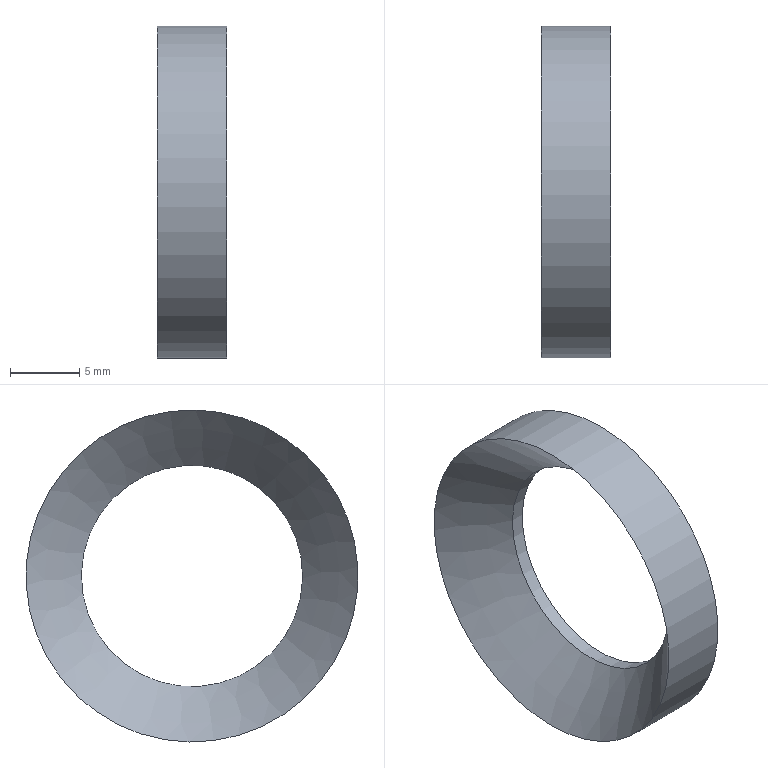Component | NX | WASHER | 1 solid | 4 faces | box 5 x 24 x 24 mm | volume 787 mm3 | cylinder 2 | plane 1 | cone 1 | commonest cylinder face diameters 24 x1 16 x1
STEP:
#1=CARTESIAN_POINT('',(0.,0.,0.));
#2=DIRECTION('',(0.,0.,1.));
#3=DIRECTION('',(1.,0.,0.));
#4=AXIS2_PLACEMENT_3D('',#1,#2,#3);
#5=CARTESIAN_POINT('',(20.,11.091,4.582));
#6=VERTEX_POINT('',#5);
#7=CARTESIAN_POINT('',(20.,0.,0.));
#8=DIRECTION('',(-1.,0.,0.));
#9=DIRECTION('',(0.,0.9242,0.3818));
#10=AXIS2_PLACEMENT_3D('',#7,#8,#9);
#11=CIRCLE('',#10,12.);
#12=CARTESIAN_POINT('',(20.,0.,0.));
#13=DIRECTION('',(1.,0.,0.));
#14=DIRECTION('',(0.,-0.9242,-0.3818));
#15=AXIS2_PLACEMENT_3D('',#12,#13,#14);
#16=CYLINDRICAL_SURFACE('',#15,12.);
#17=CARTESIAN_POINT('',(9.425,0.));
#18=DIRECTION('',(-1.,0.));
#19=VECTOR('',#18,1.);
#20=LINE('',#17,#19);
#21=(GEOMETRIC_REPRESENTATION_CONTEXT(2)PARAMETRIC_REPRESENTATION_CONTEXT()REPRESENTATION_CONTEXT('',''));
#22=DEFINITIONAL_REPRESENTATION('',(#20),#21);
#23=PCURVE('',#16,#22);
#24=CARTESIAN_POINT('',(24.,0.,0.));
#25=DIRECTION('',(-1.,0.,0.));
#26=DIRECTION('',(0.,0.9242,0.3818));
#27=AXIS2_PLACEMENT_3D('',#24,#25,#26);
#28=CONICAL_SURFACE('',#27,8.,0.7854);
#29=CARTESIAN_POINT('',(0.,4.));
#30=DIRECTION('',(1.,0.));
#31=VECTOR('',#30,1.);
#32=LINE('',#29,#31);
#33=(GEOMETRIC_REPRESENTATION_CONTEXT(2)PARAMETRIC_REPRESENTATION_CONTEXT()REPRESENTATION_CONTEXT('',''));
#34=DEFINITIONAL_REPRESENTATION('',(#32),#33);
#35=PCURVE('',#28,#34);
#36=SURFACE_CURVE('',#11,(#23,#35),.PCURVE_S1.);
#37=EDGE_CURVE('',#6,#6,#36,.T.);
#38=ORIENTED_EDGE('',*,*,#37,.F.);
#39=CARTESIAN_POINT('',(25.,11.091,4.582));
#40=VERTEX_POINT('',#39);
#41=CARTESIAN_POINT('',(20.,11.091,4.582));
#42=CARTESIAN_POINT('',(25.,11.091,4.582));
#43=B_SPLINE_CURVE_WITH_KNOTS('',1,(#41,#42),.UNSPECIFIED.,.F.,.F.,(2,2),(0.,5.),.PIECEWISE_BEZIER_KNOTS.);
#44=CARTESIAN_POINT('',(9.425,0.));
#45=DIRECTION('',(0.,1.));
#46=VECTOR('',#45,1.);
#47=LINE('',#44,#46);
#48=(GEOMETRIC_REPRESENTATION_CONTEXT(2)PARAMETRIC_REPRESENTATION_CONTEXT()REPRESENTATION_CONTEXT('',''));
#49=DEFINITIONAL_REPRESENTATION('',(#47),#48);
#50=PCURVE('',#16,#49);
#51=CARTESIAN_POINT('',(3.142,0.));
#52=DIRECTION('',(0.,1.));
#53=VECTOR('',#52,1.);
#54=LINE('',#51,#53);
#55=(GEOMETRIC_REPRESENTATION_CONTEXT(2)PARAMETRIC_REPRESENTATION_CONTEXT()REPRESENTATION_CONTEXT('',''));
#56=DEFINITIONAL_REPRESENTATION('',(#54),#55);
#57=PCURVE('',#16,#56);
#58=SEAM_CURVE('',#43,(#50,#57),.PCURVE_S1.);
#59=EDGE_CURVE('',#6,#40,#58,.T.);
#60=ORIENTED_EDGE('',*,*,#59,.T.);
#61=CARTESIAN_POINT('',(25.,0.,0.));
#62=DIRECTION('',(-1.,0.,0.));
#63=DIRECTION('',(0.,0.9242,0.3818));
#64=AXIS2_PLACEMENT_3D('',#61,#62,#63);
#65=CIRCLE('',#64,12.);
#66=CARTESIAN_POINT('',(9.425,5.));
#67=DIRECTION('',(-1.,0.));
#68=VECTOR('',#67,1.);
#69=LINE('',#66,#68);
#70=(GEOMETRIC_REPRESENTATION_CONTEXT(2)PARAMETRIC_REPRESENTATION_CONTEXT()REPRESENTATION_CONTEXT('',''));
#71=DEFINITIONAL_REPRESENTATION('',(#69),#70);
#72=PCURVE('',#16,#71);
#73=CARTESIAN_POINT('',(25.,0.,0.));
#74=DIRECTION('',(-1.,0.,0.));
#75=DIRECTION('',(0.,0.9242,0.3818));
#76=AXIS2_PLACEMENT_3D('',#73,#74,#75);
#77=PLANE('',#76);
#78=CARTESIAN_POINT('',(0.,0.));
#79=DIRECTION('',(1.,0.));
#80=AXIS2_PLACEMENT_2D('',#78,#79);
#81=CIRCLE('',#80,12.);
#82=(GEOMETRIC_REPRESENTATION_CONTEXT(2)PARAMETRIC_REPRESENTATION_CONTEXT()REPRESENTATION_CONTEXT('',''));
#83=DEFINITIONAL_REPRESENTATION('',(#81),#82);
#84=PCURVE('',#77,#83);
#85=SURFACE_CURVE('',#65,(#72,#84),.PCURVE_S1.);
#86=EDGE_CURVE('',#40,#40,#85,.T.);
#87=ORIENTED_EDGE('',*,*,#86,.T.);
#88=ORIENTED_EDGE('',*,*,#59,.F.);
#89=EDGE_LOOP('',(#38,#60,#87,#88));
#90=FACE_BOUND('',#89,.T.);
#91=ADVANCED_FACE('',(#90),#16,.T.);
#92=CARTESIAN_POINT('',(24.,7.394,3.055));
#93=VERTEX_POINT('',#92);
#94=CARTESIAN_POINT('',(24.,0.,0.));
#95=DIRECTION('',(-1.,0.,0.));
#96=DIRECTION('',(0.,0.9242,0.3818));
#97=AXIS2_PLACEMENT_3D('',#94,#95,#96);
#98=CIRCLE('',#97,8.);
#99=CARTESIAN_POINT('',(20.,0.,0.));
#100=DIRECTION('',(1.,0.,0.));
#101=DIRECTION('',(0.,-0.9242,-0.3818));
#102=AXIS2_PLACEMENT_3D('',#99,#100,#101);
#103=CYLINDRICAL_SURFACE('',#102,8.);
#104=CARTESIAN_POINT('',(9.425,4.));
#105=DIRECTION('',(-1.,0.));
#106=VECTOR('',#105,1.);
#107=LINE('',#104,#106);
#108=(GEOMETRIC_REPRESENTATION_CONTEXT(2)PARAMETRIC_REPRESENTATION_CONTEXT()REPRESENTATION_CONTEXT('',''));
#109=DEFINITIONAL_REPRESENTATION('',(#107),#108);
#110=PCURVE('',#103,#109);
#111=CARTESIAN_POINT('',(0.,0.));
#112=DIRECTION('',(1.,0.));
#113=VECTOR('',#112,1.);
#114=LINE('',#111,#113);
#115=(GEOMETRIC_REPRESENTATION_CONTEXT(2)PARAMETRIC_REPRESENTATION_CONTEXT()REPRESENTATION_CONTEXT('',''));
#116=DEFINITIONAL_REPRESENTATION('',(#114),#115);
#117=PCURVE('',#28,#116);
#118=SURFACE_CURVE('',#98,(#110,#117),.PCURVE_S1.);
#119=EDGE_CURVE('',#93,#93,#118,.T.);
#120=ORIENTED_EDGE('',*,*,#119,.F.);
#121=CARTESIAN_POINT('',(25.,7.394,3.055));
#122=VERTEX_POINT('',#121);
#123=CARTESIAN_POINT('',(24.,7.394,3.055));
#124=CARTESIAN_POINT('',(25.,7.394,3.055));
#125=B_SPLINE_CURVE_WITH_KNOTS('',1,(#123,#124),.UNSPECIFIED.,.F.,.F.,(2,2),(4.,5.),.PIECEWISE_BEZIER_KNOTS.);
#126=CARTESIAN_POINT('',(9.425,0.));
#127=DIRECTION('',(0.,1.));
#128=VECTOR('',#127,1.);
#129=LINE('',#126,#128);
#130=(GEOMETRIC_REPRESENTATION_CONTEXT(2)PARAMETRIC_REPRESENTATION_CONTEXT()REPRESENTATION_CONTEXT('',''));
#131=DEFINITIONAL_REPRESENTATION('',(#129),#130);
#132=PCURVE('',#103,#131);
#133=CARTESIAN_POINT('',(3.142,0.));
#134=DIRECTION('',(0.,1.));
#135=VECTOR('',#134,1.);
#136=LINE('',#133,#135);
#137=(GEOMETRIC_REPRESENTATION_CONTEXT(2)PARAMETRIC_REPRESENTATION_CONTEXT()REPRESENTATION_CONTEXT('',''));
#138=DEFINITIONAL_REPRESENTATION('',(#136),#137);
#139=PCURVE('',#103,#138);
#140=SEAM_CURVE('',#125,(#132,#139),.PCURVE_S1.);
#141=EDGE_CURVE('',#93,#122,#140,.T.);
#142=ORIENTED_EDGE('',*,*,#141,.T.);
#143=CARTESIAN_POINT('',(25.,0.,0.));
#144=DIRECTION('',(-1.,0.,0.));
#145=DIRECTION('',(0.,0.9242,0.3818));
#146=AXIS2_PLACEMENT_3D('',#143,#144,#145);
#147=CIRCLE('',#146,8.);
#148=CARTESIAN_POINT('',(9.425,5.));
#149=DIRECTION('',(-1.,0.));
#150=VECTOR('',#149,1.);
#151=LINE('',#148,#150);
#152=(GEOMETRIC_REPRESENTATION_CONTEXT(2)PARAMETRIC_REPRESENTATION_CONTEXT()REPRESENTATION_CONTEXT('',''));
#153=DEFINITIONAL_REPRESENTATION('',(#151),#152);
#154=PCURVE('',#103,#153);
#155=CARTESIAN_POINT('',(0.,0.));
#156=DIRECTION('',(1.,0.));
#157=AXIS2_PLACEMENT_2D('',#155,#156);
#158=CIRCLE('',#157,8.);
#159=(GEOMETRIC_REPRESENTATION_CONTEXT(2)PARAMETRIC_REPRESENTATION_CONTEXT()REPRESENTATION_CONTEXT('',''));
#160=DEFINITIONAL_REPRESENTATION('',(#158),#159);
#161=PCURVE('',#77,#160);
#162=SURFACE_CURVE('',#147,(#154,#161),.PCURVE_S1.);
#163=EDGE_CURVE('',#122,#122,#162,.T.);
#164=ORIENTED_EDGE('',*,*,#163,.T.);
#165=ORIENTED_EDGE('',*,*,#141,.F.);
#166=EDGE_LOOP('',(#120,#142,#164,#165));
#167=FACE_BOUND('',#166,.F.);
#168=ADVANCED_FACE('',(#167),#103,.F.);
#169=ORIENTED_EDGE('',*,*,#86,.F.);
#170=EDGE_LOOP('',(#169));
#171=FACE_BOUND('',#170,.T.);
#172=ORIENTED_EDGE('',*,*,#163,.T.);
#173=EDGE_LOOP('',(#172));
#174=FACE_BOUND('',#173,.T.);
#175=ADVANCED_FACE('',(#171,#174),#77,.F.);
#176=ORIENTED_EDGE('',*,*,#37,.F.);
#177=CARTESIAN_POINT('',(24.,7.394,3.055));
#178=CARTESIAN_POINT('',(20.,11.091,4.582));
#179=B_SPLINE_CURVE_WITH_KNOTS('',1,(#177,#178),.UNSPECIFIED.,.F.,.F.,(2,2),(0.,5.657),.PIECEWISE_BEZIER_KNOTS.);
#180=CARTESIAN_POINT('',(0.,0.));
#181=DIRECTION('',(0.,1.));
#182=VECTOR('',#181,1.);
#183=LINE('',#180,#182);
#184=(GEOMETRIC_REPRESENTATION_CONTEXT(2)PARAMETRIC_REPRESENTATION_CONTEXT()REPRESENTATION_CONTEXT('',''));
#185=DEFINITIONAL_REPRESENTATION('',(#183),#184);
#186=PCURVE('',#28,#185);
#187=CARTESIAN_POINT('',(6.283,0.));
#188=DIRECTION('',(0.,1.));
#189=VECTOR('',#188,1.);
#190=LINE('',#187,#189);
#191=(GEOMETRIC_REPRESENTATION_CONTEXT(2)PARAMETRIC_REPRESENTATION_CONTEXT()REPRESENTATION_CONTEXT('',''));
#192=DEFINITIONAL_REPRESENTATION('',(#190),#191);
#193=PCURVE('',#28,#192);
#194=SEAM_CURVE('',#179,(#186,#193),.PCURVE_S1.);
#195=EDGE_CURVE('',#93,#6,#194,.T.);
#196=ORIENTED_EDGE('',*,*,#195,.F.);
#197=ORIENTED_EDGE('',*,*,#119,.T.);
#198=ORIENTED_EDGE('',*,*,#195,.T.);
#199=EDGE_LOOP('',(#176,#196,#197,#198));
#200=FACE_BOUND('',#199,.F.);
#201=ADVANCED_FACE('',(#200),#28,.F.);
#202=CLOSED_SHELL('',(#91,#168,#175,#201));
#203=MANIFOLD_SOLID_BREP('',#202);
#204=(LENGTH_UNIT()NAMED_UNIT(*)SI_UNIT(.MILLI.,.METRE.));
#205=UNCERTAINTY_MEASURE_WITH_UNIT(LENGTH_MEASURE(0.00001),#204,'','');
#206=(NAMED_UNIT(*)PLANE_ANGLE_UNIT()SI_UNIT($,.RADIAN.));
#207=(NAMED_UNIT(*)SI_UNIT($,.STERADIAN.)SOLID_ANGLE_UNIT());
#208=(GEOMETRIC_REPRESENTATION_CONTEXT(3)GLOBAL_UNCERTAINTY_ASSIGNED_CONTEXT((#205))GLOBAL_UNIT_ASSIGNED_CONTEXT((#204,#206,#207))REPRESENTATION_CONTEXT('',''));
#209=ADVANCED_BREP_SHAPE_REPRESENTATION('',(#4,#203),#208);